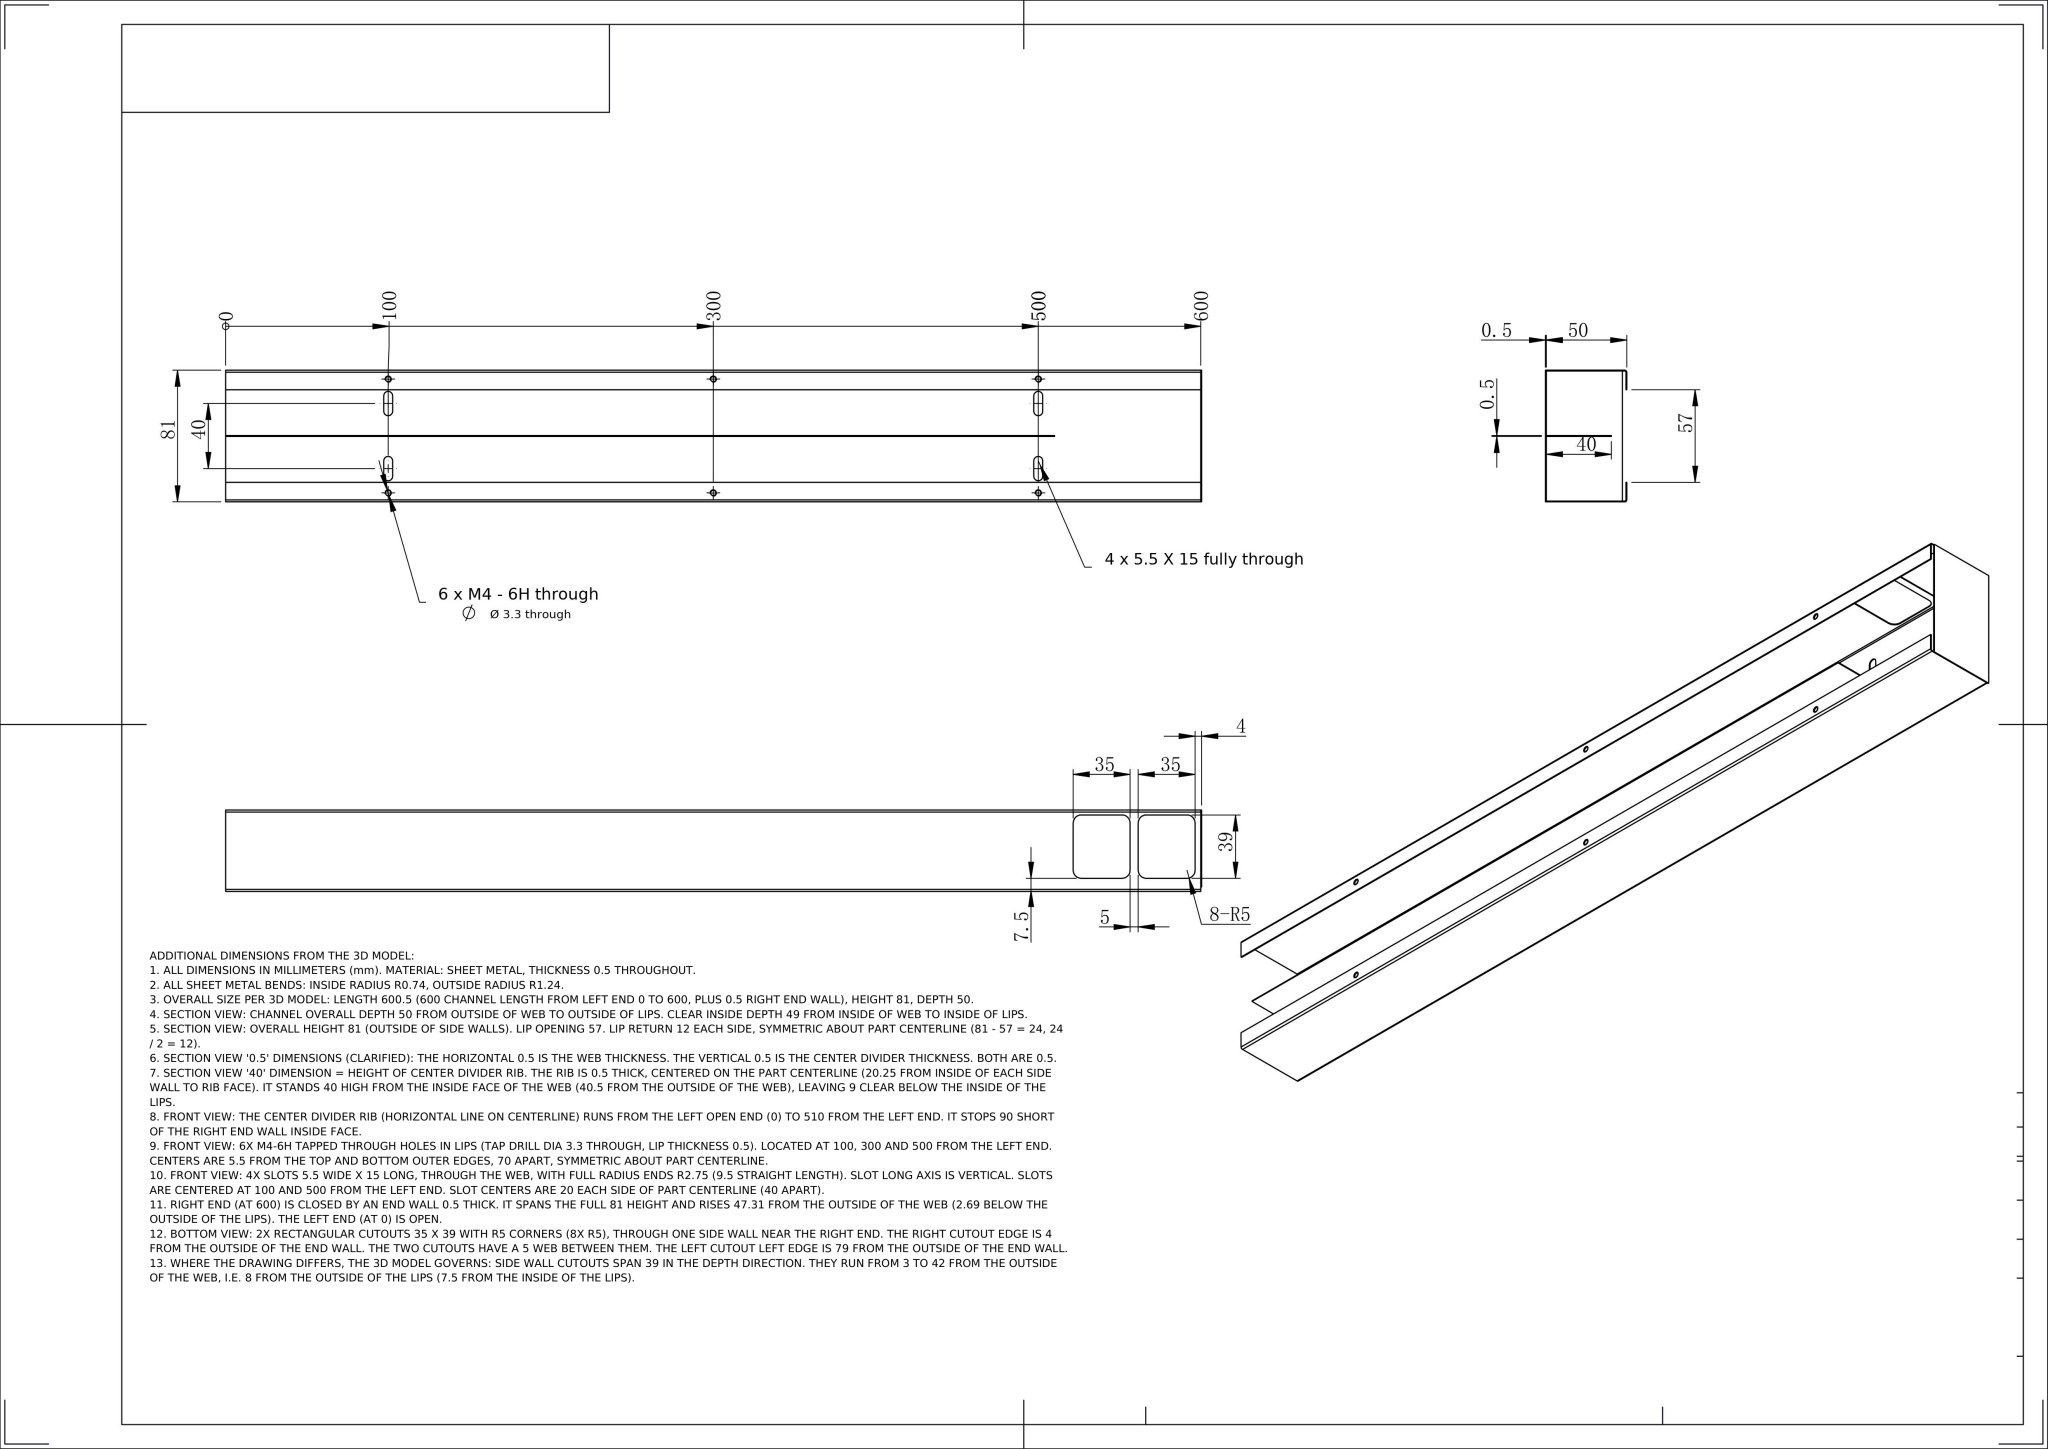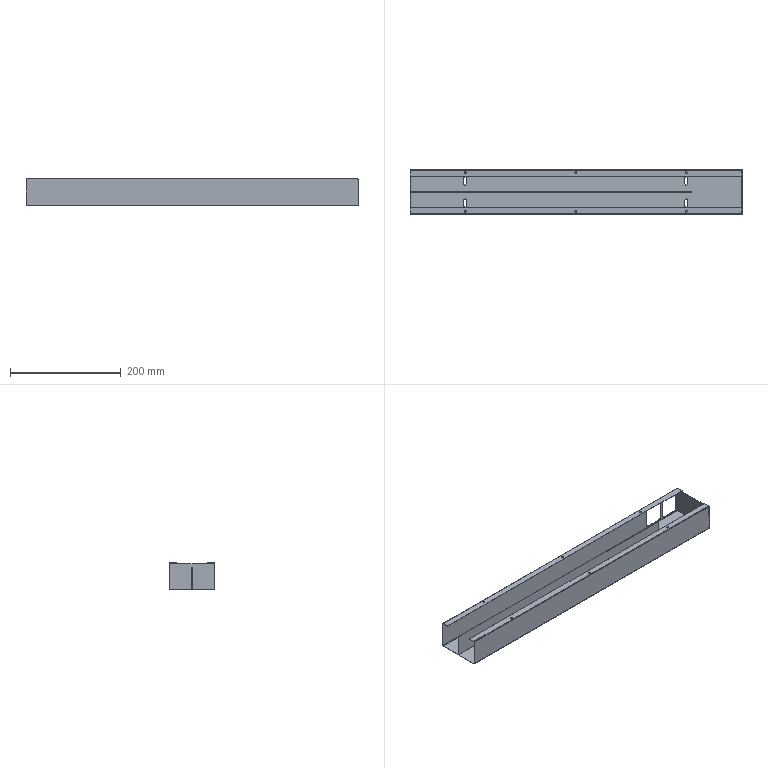Part | NX | mm | 1 solid | 88 faces | box 600.5 x 81 x 50 mm | volume 70987 mm3 | plane 52 | cylinder 36 | commonest cylinder face diameters 3.3 x12 10 x8 5.5 x8 1.473 x4 2.473 x4